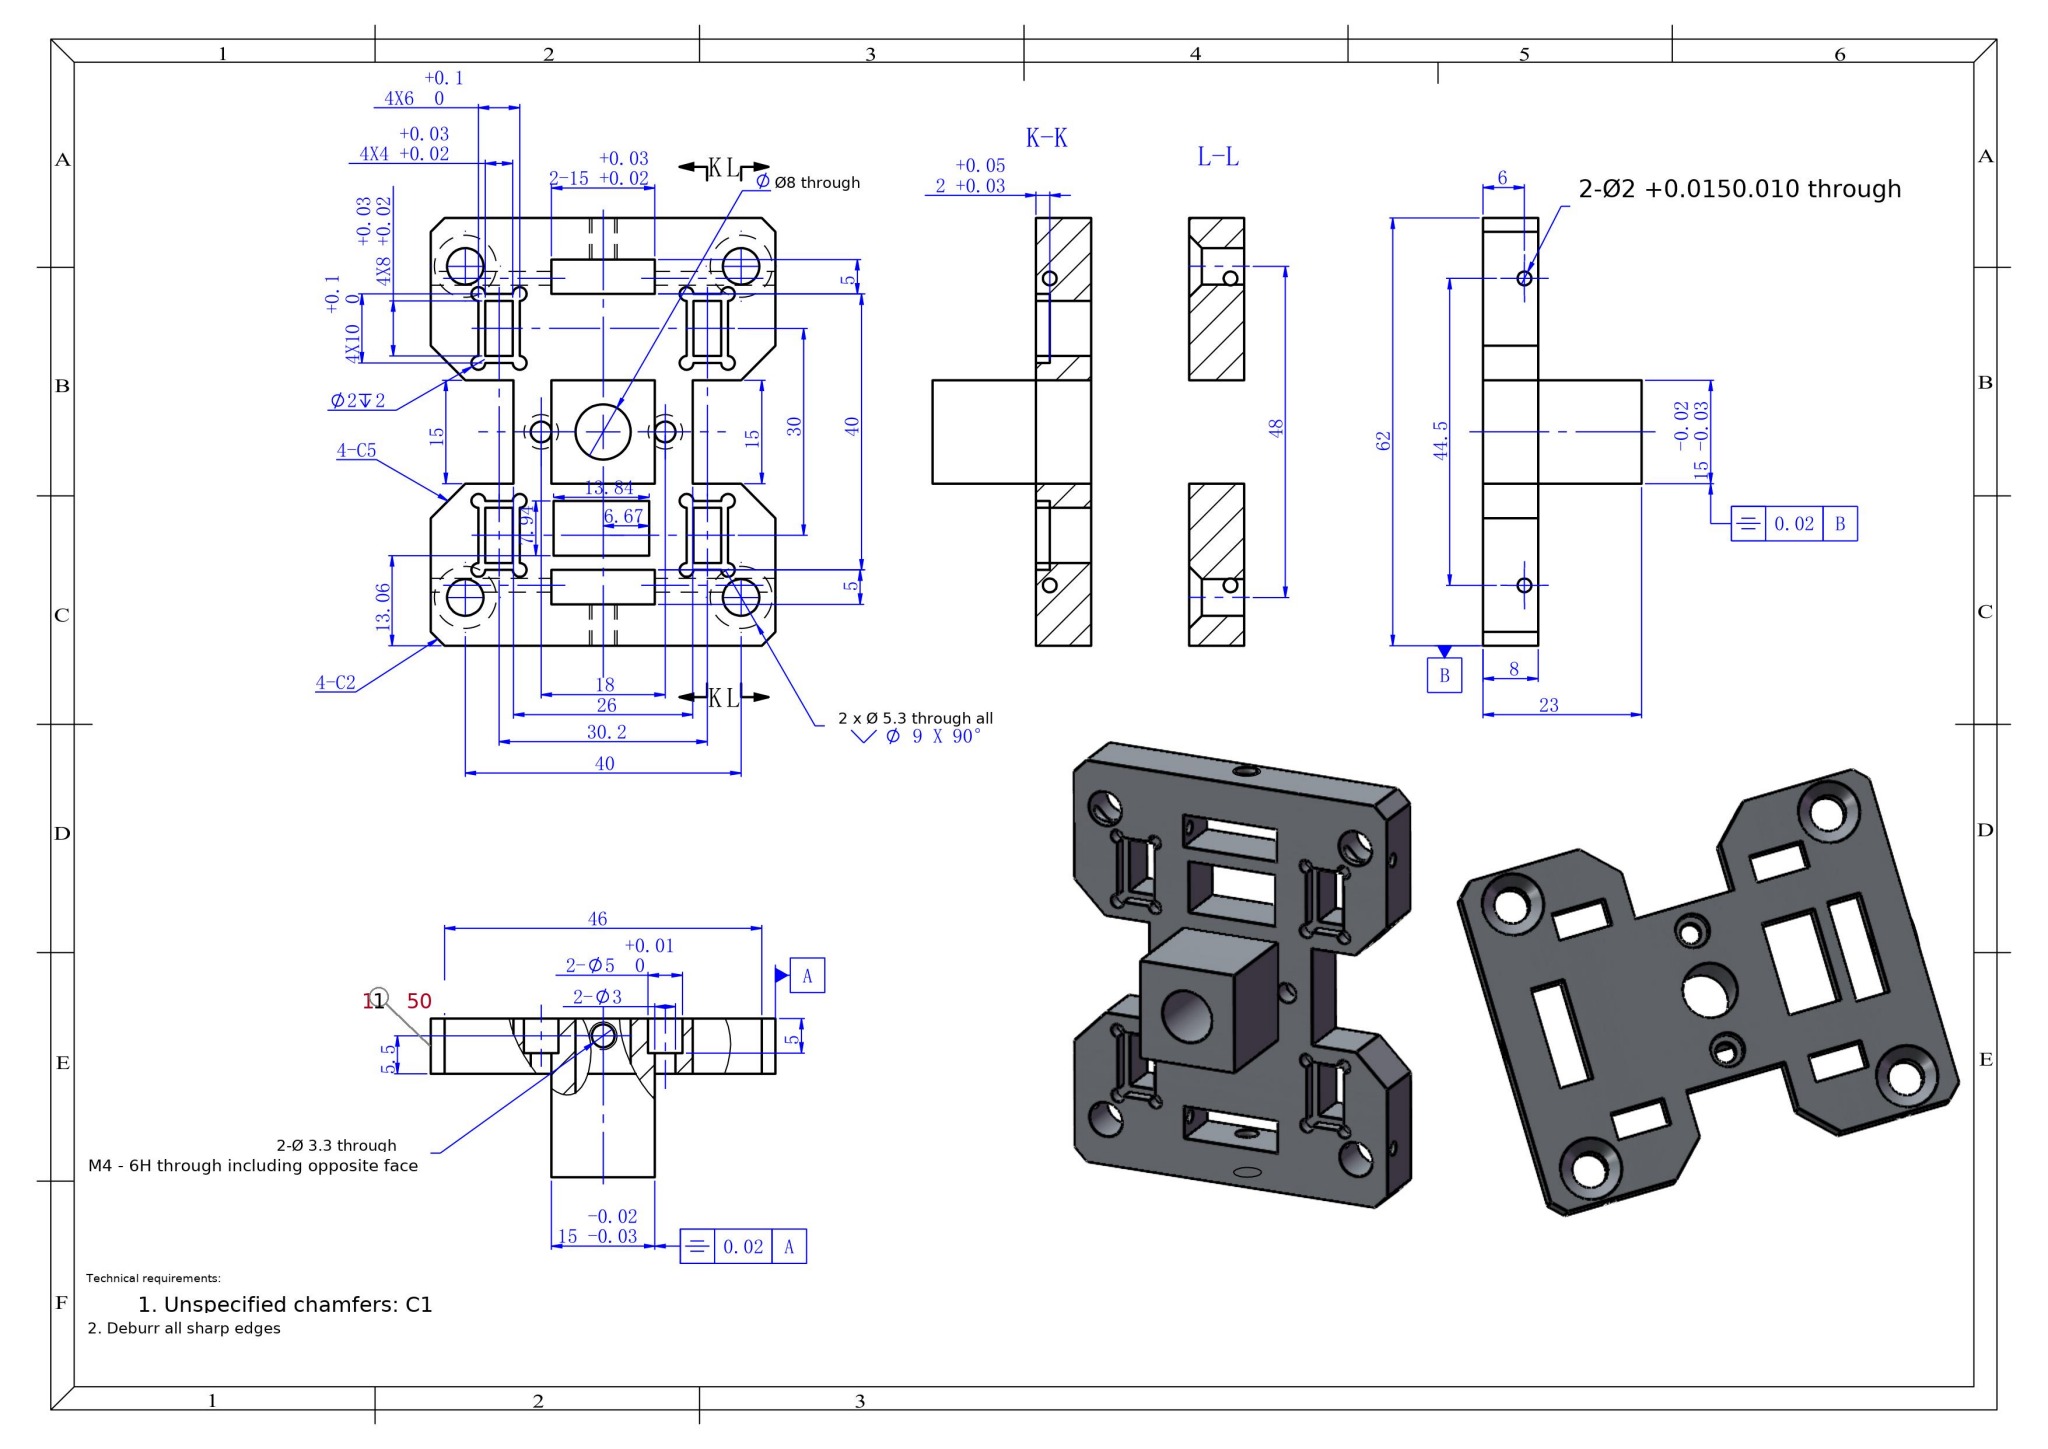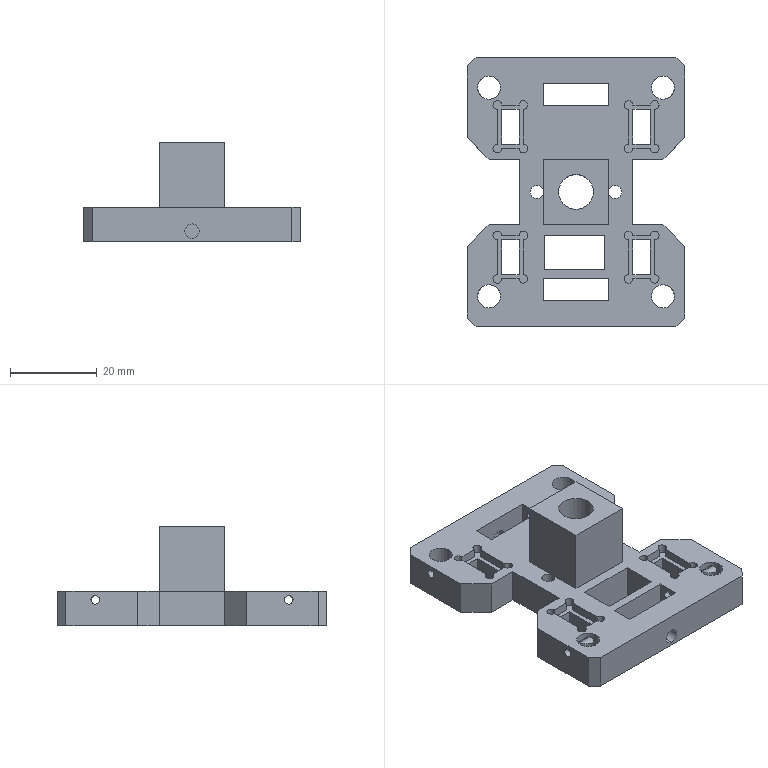Part | SolidWorks | 1 solid | 139 faces | box 50 x 62 x 23 mm | volume 18911 mm3 | plane 77 | cylinder 54 | cone 8 | commonest cylinder face diameters 2 x32 5.3 x8 3 x4 5 x4 3.3 x4 8 x2